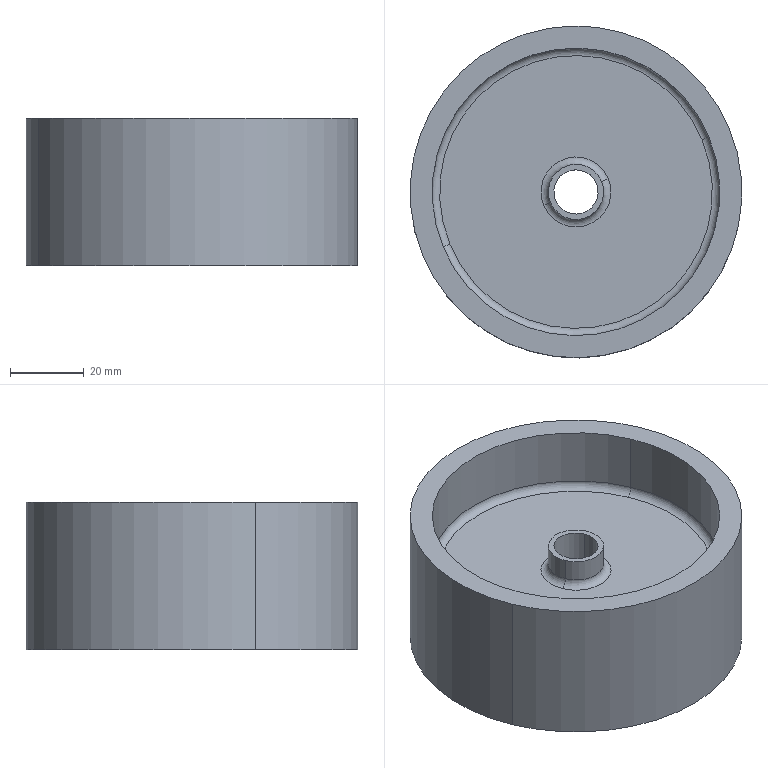Component | SolidWorks | SpringCover-2 | 1 solid | 38 faces | box 90 x 90 x 40 mm | volume 80853 mm3 | cylinder 18 | torus 12 | plane 8 | commonest cylinder face diameters 78 x4 82 x2 15 x2 86 x2 18 x2 24 x2 12 x2 90 x2
build123d program:
from build123d import *

# Parameters (mm, degrees)
SKETCH1_2_R         = 45
SKETCH1_2_R_2       = 39
BOSS_EXTRUDE1_DEPTH = 20
SKETCH2_R           = 40
SKETCH2_R_2         = 6
BOSS_EXTRUDE2_DEPTH = 2
SKETCH3_R           = 12
SKETCH3_R_2         = 9
BOSS_EXTRUDE3_DEPTH = 16
BOSS_EXTRUDE4_START = 8
SKETCH5_R           = 7.5
SKETCH5_R_2         = 6
BOSS_EXTRUDE4_DEPTH = 8
FILLET1_R           = 2
CUT_EXTRUDE1_START  = -6
SKETCH1_R           = 43
SKETCH1_R_2         = 41
CUT_EXTRUDE1_DEPTH  = 6


with BuildPart() as part:
    # Sketch1_2 → Boss-Extrude1 (new, symmetric)
    with BuildSketch(Plane.XY):
        Circle(SKETCH1_2_R)
        Circle(SKETCH1_2_R_2, mode=Mode.SUBTRACT)
    extrude(amount=BOSS_EXTRUDE1_DEPTH, both=True)

    # Sketch2 → Boss-Extrude2 (add, symmetric)
    with BuildSketch(Plane.XY):
        Circle(SKETCH2_R)
        Circle(SKETCH2_R_2, mode=Mode.SUBTRACT)
    extrude(amount=BOSS_EXTRUDE2_DEPTH, both=True)

    # Sketch3 → Boss-Extrude3 (add)
    with BuildSketch(Plane.XY.offset(2)):
        Circle(SKETCH3_R)
        Circle(SKETCH3_R_2, mode=Mode.SUBTRACT)
    extrude(amount=BOSS_EXTRUDE3_DEPTH)

    # Sketch4 → Cut-Revolve1 (revolve, cut)
    with BuildSketch(Plane(origin=(0, 0, 0), x_dir=(1, 0, 0), z_dir=(0, 1, 0))):
        Polygon((-43, -16), (-33.035, -16), (-33.287, -20), (-43, -20), align=None)
    revolve(axis=Axis((0, 0, -26.979), (0, 0, 1)), mode=Mode.SUBTRACT)

    # Sketch5 → Boss-Extrude4 (add)
    with BuildSketch(Plane(origin=(0, 0, -2), x_dir=(-1, 0, 0), z_dir=(0, 0, -1)).offset(BOSS_EXTRUDE4_START)):
        with Locations(Location((0, 0, 0), (0, 0, 180))):
            Circle(SKETCH5_R)
        Circle(SKETCH5_R_2, mode=Mode.SUBTRACT)
    extrude(amount=-BOSS_EXTRUDE4_DEPTH)

    # Fillet1
    fillet1_edges = [part.edges().sort_by_distance(p)[0] for p in [
        (-39, 0, 2),
        (-39, 0, -2),
        (-9, 0, 2),
        (-12, 0, 2),
        (-39, 0, 16),
        (-7.5, 0, -2),
    ]]
    fillet(fillet1_edges, radius=FILLET1_R)

    # Sketch1 → Cut-Extrude1 (cut)
    with BuildSketch(Plane.XY.offset(20).offset(CUT_EXTRUDE1_START)):
        with Locations(Location((0, 0, 0), (0, 0, 180))):
            Circle(SKETCH1_R)
        Circle(SKETCH1_R_2, mode=Mode.SUBTRACT)
    extrude(amount=CUT_EXTRUDE1_DEPTH, mode=Mode.SUBTRACT)


solid = part.part

# Placed as in the assembly
solid = solid.moved(Location((-15.928, -1.7, 188), (180, 0, 0)))
STEP:
#1=COLOUR_RGB('',0.7922,0.8196,0.9333);
#2=FILL_AREA_STYLE_COLOUR('',#1);
#3=FILL_AREA_STYLE('',(#2));
#4=SURFACE_STYLE_FILL_AREA(#3);
#5=SURFACE_SIDE_STYLE('',(#4));
#6=SURFACE_STYLE_USAGE(.BOTH.,#5);
#7=PRESENTATION_STYLE_ASSIGNMENT((#6));
#8=CARTESIAN_POINT('',(0.864,0.5514,6.85));
#9=VERTEX_POINT('',#8);
#10=CARTESIAN_POINT('',(-2.118,-0.6852,6.85));
#11=VERTEX_POINT('',#10);
#12=CARTESIAN_POINT('',(-0.6271,-0.06694,6.85));
#13=DIRECTION('',(0.,0.,-1.));
#14=DIRECTION('',(0.9237,0.383,0.));
#15=AXIS2_PLACEMENT_3D('',#12,#13,#14);
#16=CIRCLE('',#15,1.614);
#17=EDGE_CURVE('',#9,#11,#16,.T.);
#18=ORIENTED_EDGE('',*,*,#17,.T.);
#19=CARTESIAN_POINT('',(-2.118,-0.6852,6.772));
#20=VERTEX_POINT('',#19);
#21=CARTESIAN_POINT('',(-2.118,-0.6852,6.85));
#22=DIRECTION('',(0.,0.,-1.));
#23=VECTOR('',#22,39.37);
#24=LINE('',#21,#23);
#25=EDGE_CURVE('',#11,#20,#24,.T.);
#26=ORIENTED_EDGE('',*,*,#25,.T.);
#27=CARTESIAN_POINT('',(0.864,0.5514,6.772));
#28=VERTEX_POINT('',#27);
#29=CARTESIAN_POINT('',(-0.6271,-0.06694,6.772));
#30=DIRECTION('',(0.,0.,-1.));
#31=DIRECTION('',(-0.9237,-0.383,0.));
#32=AXIS2_PLACEMENT_3D('',#29,#30,#31);
#33=CIRCLE('',#32,1.614);
#34=EDGE_CURVE('',#28,#20,#33,.T.);
#35=ORIENTED_EDGE('',*,*,#34,.F.);
#36=CARTESIAN_POINT('',(0.864,0.5514,6.85));
#37=DIRECTION('',(0.,0.,-1.));
#38=VECTOR('',#37,39.37);
#39=LINE('',#36,#38);
#40=EDGE_CURVE('',#9,#28,#39,.T.);
#41=ORIENTED_EDGE('',*,*,#40,.F.);
#42=EDGE_LOOP('',(#18,#26,#35,#41));
#43=FACE_OUTER_BOUND('',#42,.T.);
#44=CARTESIAN_POINT('',(-0.6271,-0.06694,6.85));
#45=DIRECTION('',(0.,0.,-1.));
#46=DIRECTION('',(0.9237,0.383,0.));
#47=AXIS2_PLACEMENT_3D('',#44,#45,#46);
#48=CYLINDRICAL_SURFACE('',#47,1.614);
#49=ADVANCED_FACE('',(#43),#48,.T.);
#50=CARTESIAN_POINT('',(-1.973,-0.6249,7.323));
#51=VERTEX_POINT('',#50);
#52=CARTESIAN_POINT('',(0.7185,0.491,7.323));
#53=VERTEX_POINT('',#52);
#54=CARTESIAN_POINT('',(-0.6271,-0.06694,7.323));
#55=DIRECTION('',(0.,0.,-1.));
#56=DIRECTION('',(0.9237,0.383,0.));
#57=AXIS2_PLACEMENT_3D('',#54,#55,#56);
#58=CIRCLE('',#57,1.457);
#59=EDGE_CURVE('',#51,#53,#58,.T.);
#60=ORIENTED_EDGE('',*,*,#59,.F.);
#61=CARTESIAN_POINT('',(-2.045,-0.6551,7.244));
#62=VERTEX_POINT('',#61);
#63=CARTESIAN_POINT('',(-1.973,-0.6249,7.244));
#64=DIRECTION('',(0.383,-0.9237,0.));
#65=DIRECTION('',(0.9237,0.383,0.));
#66=AXIS2_PLACEMENT_3D('',#63,#64,#65);
#67=CIRCLE('',#66,0.07874);
#68=EDGE_CURVE('',#51,#62,#67,.T.);
#69=ORIENTED_EDGE('',*,*,#68,.T.);
#70=CARTESIAN_POINT('',(0.7912,0.5212,7.244));
#71=VERTEX_POINT('',#70);
#72=CARTESIAN_POINT('',(-0.6271,-0.06694,7.244));
#73=DIRECTION('',(0.,0.,1.));
#74=DIRECTION('',(0.9237,0.383,0.));
#75=AXIS2_PLACEMENT_3D('',#72,#73,#74);
#76=CIRCLE('',#75,1.535);
#77=EDGE_CURVE('',#71,#62,#76,.T.);
#78=ORIENTED_EDGE('',*,*,#77,.F.);
#79=CARTESIAN_POINT('',(0.7185,0.491,7.244));
#80=DIRECTION('',(-0.383,0.9237,0.));
#81=DIRECTION('',(-0.9237,-0.383,0.));
#82=AXIS2_PLACEMENT_3D('',#79,#80,#81);
#83=CIRCLE('',#82,0.07874);
#84=EDGE_CURVE('',#53,#71,#83,.T.);
#85=ORIENTED_EDGE('',*,*,#84,.F.);
#86=EDGE_LOOP('',(#60,#69,#78,#85));
#87=FACE_OUTER_BOUND('',#86,.T.);
#88=CARTESIAN_POINT('',(-0.6271,-0.06694,7.244));
#89=DIRECTION('',(0.,0.,-1.));
#90=DIRECTION('',(0.9237,0.383,0.));
#91=AXIS2_PLACEMENT_3D('',#88,#89,#90);
#92=TOROIDAL_SURFACE('',#91,1.457,0.07874);
#93=ADVANCED_FACE('',(#87),#92,.F.);
#94=CARTESIAN_POINT('',(0.7912,0.5212,6.85));
#95=VERTEX_POINT('',#94);
#96=CARTESIAN_POINT('',(-2.045,-0.6551,6.85));
#97=VERTEX_POINT('',#96);
#98=CARTESIAN_POINT('',(-0.6271,-0.06694,6.85));
#99=DIRECTION('',(0.,0.,-1.));
#100=DIRECTION('',(-0.9237,-0.383,0.));
#101=AXIS2_PLACEMENT_3D('',#98,#99,#100);
#102=CIRCLE('',#101,1.535);
#103=EDGE_CURVE('',#95,#97,#102,.T.);
#104=ORIENTED_EDGE('',*,*,#103,.F.);
#105=CARTESIAN_POINT('',(0.864,0.5514,6.85));
#106=DIRECTION('',(0.383,-0.9237,0.));
#107=DIRECTION('',(0.9237,0.383,0.));
#108=AXIS2_PLACEMENT_3D('',#105,#106,#107);
#109=CIRCLE('',#108,0.07874);
#110=EDGE_CURVE('',#95,#28,#109,.T.);
#111=ORIENTED_EDGE('',*,*,#110,.T.);
#112=ORIENTED_EDGE('',*,*,#34,.T.);
#113=CARTESIAN_POINT('',(-2.118,-0.6852,6.85));
#114=DIRECTION('',(-0.383,0.9237,0.));
#115=DIRECTION('',(-0.9237,-0.383,0.));
#116=AXIS2_PLACEMENT_3D('',#113,#114,#115);
#117=CIRCLE('',#116,0.07874);
#118=EDGE_CURVE('',#97,#20,#117,.T.);
#119=ORIENTED_EDGE('',*,*,#118,.F.);
#120=EDGE_LOOP('',(#104,#111,#112,#119));
#121=FACE_OUTER_BOUND('',#120,.T.);
#122=CARTESIAN_POINT('',(-0.6271,-0.06694,6.85));
#123=DIRECTION('',(0.,0.,1.));
#124=DIRECTION('',(-0.9237,-0.383,0.));
#125=AXIS2_PLACEMENT_3D('',#122,#123,#124);
#126=TOROIDAL_SURFACE('',#125,1.614,0.07874);
#127=ADVANCED_FACE('',(#121),#126,.T.);
#128=CARTESIAN_POINT('',(-0.8817,-0.1725,7.323));
#129=VERTEX_POINT('',#128);
#130=CARTESIAN_POINT('',(-0.3725,0.03863,7.323));
#131=VERTEX_POINT('',#130);
#132=CARTESIAN_POINT('',(-0.6271,-0.06694,7.323));
#133=DIRECTION('',(0.,0.,-1.));
#134=DIRECTION('',(0.9237,0.383,0.));
#135=AXIS2_PLACEMENT_3D('',#132,#133,#134);
#136=CIRCLE('',#135,0.2756);
#137=EDGE_CURVE('',#129,#131,#136,.T.);
#138=ORIENTED_EDGE('',*,*,#137,.F.);
#139=CARTESIAN_POINT('',(-0.9544,-0.2027,7.244));
#140=VERTEX_POINT('',#139);
#141=CARTESIAN_POINT('',(-0.8817,-0.1725,7.244));
#142=DIRECTION('',(0.383,-0.9237,0.));
#143=DIRECTION('',(0.9237,0.383,0.));
#144=AXIS2_PLACEMENT_3D('',#141,#142,#143);
#145=CIRCLE('',#144,0.07874);
#146=EDGE_CURVE('',#129,#140,#145,.T.);
#147=ORIENTED_EDGE('',*,*,#146,.T.);
#148=CARTESIAN_POINT('',(-0.2998,0.06879,7.244));
#149=VERTEX_POINT('',#148);
#150=CARTESIAN_POINT('',(-0.6271,-0.06694,7.244));
#151=DIRECTION('',(0.,0.,1.));
#152=DIRECTION('',(0.9237,0.383,0.));
#153=AXIS2_PLACEMENT_3D('',#150,#151,#152);
#154=CIRCLE('',#153,0.3543);
#155=EDGE_CURVE('',#149,#140,#154,.T.);
#156=ORIENTED_EDGE('',*,*,#155,.F.);
#157=CARTESIAN_POINT('',(-0.3725,0.03863,7.244));
#158=DIRECTION('',(-0.383,0.9237,0.));
#159=DIRECTION('',(-0.9237,-0.383,0.));
#160=AXIS2_PLACEMENT_3D('',#157,#158,#159);
#161=CIRCLE('',#160,0.07874);
#162=EDGE_CURVE('',#131,#149,#161,.T.);
#163=ORIENTED_EDGE('',*,*,#162,.F.);
#164=EDGE_LOOP('',(#138,#147,#156,#163));
#165=FACE_OUTER_BOUND('',#164,.T.);
#166=CARTESIAN_POINT('',(-0.6271,-0.06694,7.244));
#167=DIRECTION('',(0.,0.,-1.));
#168=DIRECTION('',(0.9237,0.383,0.));
#169=AXIS2_PLACEMENT_3D('',#166,#167,#168);
#170=TOROIDAL_SURFACE('',#169,0.2756,0.07874);
#171=ADVANCED_FACE('',(#165),#170,.F.);
#172=CARTESIAN_POINT('',(-1.063,-0.2479,7.244));
#173=VERTEX_POINT('',#172);
#174=CARTESIAN_POINT('',(-0.1907,0.114,7.244));
#175=VERTEX_POINT('',#174);
#176=CARTESIAN_POINT('',(-0.6271,-0.06694,7.244));
#177=DIRECTION('',(0.,0.,-1.));
#178=DIRECTION('',(0.9237,0.383,0.));
#179=AXIS2_PLACEMENT_3D('',#176,#177,#178);
#180=CIRCLE('',#179,0.4724);
#181=EDGE_CURVE('',#173,#175,#180,.T.);
#182=ORIENTED_EDGE('',*,*,#181,.F.);
#183=CARTESIAN_POINT('',(-1.136,-0.2781,7.323));
#184=VERTEX_POINT('',#183);
#185=CARTESIAN_POINT('',(-1.136,-0.2781,7.244));
#186=DIRECTION('',(0.383,-0.9237,0.));
#187=DIRECTION('',(0.9237,0.383,0.));
#188=AXIS2_PLACEMENT_3D('',#185,#186,#187);
#189=CIRCLE('',#188,0.07874);
#190=EDGE_CURVE('',#173,#184,#189,.T.);
#191=ORIENTED_EDGE('',*,*,#190,.T.);
#192=CARTESIAN_POINT('',(-0.1179,0.1442,7.323));
#193=VERTEX_POINT('',#192);
#194=CARTESIAN_POINT('',(-0.6271,-0.06694,7.323));
#195=DIRECTION('',(0.,0.,1.));
#196=DIRECTION('',(0.9237,0.383,0.));
#197=AXIS2_PLACEMENT_3D('',#194,#195,#196);
#198=CIRCLE('',#197,0.5512);
#199=EDGE_CURVE('',#193,#184,#198,.T.);
#200=ORIENTED_EDGE('',*,*,#199,.F.);
#201=CARTESIAN_POINT('',(-0.1179,0.1442,7.244));
#202=DIRECTION('',(-0.383,0.9237,0.));
#203=DIRECTION('',(-0.9237,-0.383,0.));
#204=AXIS2_PLACEMENT_3D('',#201,#202,#203);
#205=CIRCLE('',#204,0.07874);
#206=EDGE_CURVE('',#175,#193,#205,.T.);
#207=ORIENTED_EDGE('',*,*,#206,.F.);
#208=EDGE_LOOP('',(#182,#191,#200,#207));
#209=FACE_OUTER_BOUND('',#208,.T.);
#210=CARTESIAN_POINT('',(-0.6271,-0.06694,7.244));
#211=DIRECTION('',(0.,0.,-1.));
#212=DIRECTION('',(0.9237,0.383,0.));
#213=AXIS2_PLACEMENT_3D('',#210,#211,#212);
#214=TOROIDAL_SURFACE('',#213,0.5512,0.07874);
#215=ADVANCED_FACE('',(#209),#214,.F.);
#216=CARTESIAN_POINT('',(-2.045,-0.6551,7.559));
#217=VERTEX_POINT('',#216);
#218=CARTESIAN_POINT('',(0.7912,0.5212,7.559));
#219=VERTEX_POINT('',#218);
#220=CARTESIAN_POINT('',(-0.6271,-0.06694,7.559));
#221=DIRECTION('',(0.,0.,-1.));
#222=DIRECTION('',(0.9237,0.383,0.));
#223=AXIS2_PLACEMENT_3D('',#220,#221,#222);
#224=CIRCLE('',#223,1.535);
#225=EDGE_CURVE('',#217,#219,#224,.T.);
#226=ORIENTED_EDGE('',*,*,#225,.F.);
#227=CARTESIAN_POINT('',(-1.973,-0.6249,7.48));
#228=VERTEX_POINT('',#227);
#229=CARTESIAN_POINT('',(-1.973,-0.6249,7.559));
#230=DIRECTION('',(0.383,-0.9237,0.));
#231=DIRECTION('',(0.9237,0.383,0.));
#232=AXIS2_PLACEMENT_3D('',#229,#230,#231);
#233=CIRCLE('',#232,0.07874);
#234=EDGE_CURVE('',#217,#228,#233,.T.);
#235=ORIENTED_EDGE('',*,*,#234,.T.);
#236=CARTESIAN_POINT('',(0.7185,0.491,7.48));
#237=VERTEX_POINT('',#236);
#238=CARTESIAN_POINT('',(-0.6271,-0.06694,7.48));
#239=DIRECTION('',(0.,0.,1.));
#240=DIRECTION('',(0.9237,0.383,0.));
#241=AXIS2_PLACEMENT_3D('',#238,#239,#240);
#242=CIRCLE('',#241,1.457);
#243=EDGE_CURVE('',#237,#228,#242,.T.);
#244=ORIENTED_EDGE('',*,*,#243,.F.);
#245=CARTESIAN_POINT('',(0.7185,0.491,7.559));
#246=DIRECTION('',(-0.383,0.9237,0.));
#247=DIRECTION('',(-0.9237,-0.383,0.));
#248=AXIS2_PLACEMENT_3D('',#245,#246,#247);
#249=CIRCLE('',#248,0.07874);
#250=EDGE_CURVE('',#219,#237,#249,.T.);
#251=ORIENTED_EDGE('',*,*,#250,.F.);
#252=EDGE_LOOP('',(#226,#235,#244,#251));
#253=FACE_OUTER_BOUND('',#252,.T.);
#254=CARTESIAN_POINT('',(-0.6271,-0.06694,7.559));
#255=DIRECTION('',(0.,0.,-1.));
#256=DIRECTION('',(0.9237,0.383,0.));
#257=AXIS2_PLACEMENT_3D('',#254,#255,#256);
#258=TOROIDAL_SURFACE('',#257,1.457,0.07874);
#259=ADVANCED_FACE('',(#253),#258,.F.);
#260=CARTESIAN_POINT('',(-0.9726,-0.2102,7.48));
#261=VERTEX_POINT('',#260);
#262=CARTESIAN_POINT('',(-0.2816,0.07633,7.48));
#263=VERTEX_POINT('',#262);
#264=CARTESIAN_POINT('',(-0.6271,-0.06694,7.48));
#265=DIRECTION('',(0.,0.,-1.));
#266=DIRECTION('',(0.9237,0.383,0.));
#267=AXIS2_PLACEMENT_3D('',#264,#265,#266);
#268=CIRCLE('',#267,0.374);
#269=EDGE_CURVE('',#261,#263,#268,.T.);
#270=ORIENTED_EDGE('',*,*,#269,.F.);
#271=CARTESIAN_POINT('',(-0.8998,-0.18,7.559));
#272=VERTEX_POINT('',#271);
#273=CARTESIAN_POINT('',(-0.9726,-0.2102,7.559));
#274=DIRECTION('',(0.383,-0.9237,0.));
#275=DIRECTION('',(0.9237,0.383,0.));
#276=AXIS2_PLACEMENT_3D('',#273,#274,#275);
#277=CIRCLE('',#276,0.07874);
#278=EDGE_CURVE('',#261,#272,#277,.T.);
#279=ORIENTED_EDGE('',*,*,#278,.T.);
#280=CARTESIAN_POINT('',(-0.3543,0.04617,7.559));
#281=VERTEX_POINT('',#280);
#282=CARTESIAN_POINT('',(-0.6271,-0.06694,7.559));
#283=DIRECTION('',(0.,0.,1.));
#284=DIRECTION('',(0.9237,0.383,0.));
#285=AXIS2_PLACEMENT_3D('',#282,#283,#284);
#286=CIRCLE('',#285,0.2953);
#287=EDGE_CURVE('',#281,#272,#286,.T.);
#288=ORIENTED_EDGE('',*,*,#287,.F.);
#289=CARTESIAN_POINT('',(-0.2816,0.07633,7.559));
#290=DIRECTION('',(-0.383,0.9237,0.));
#291=DIRECTION('',(-0.9237,-0.383,0.));
#292=AXIS2_PLACEMENT_3D('',#289,#290,#291);
#293=CIRCLE('',#292,0.07874);
#294=EDGE_CURVE('',#263,#281,#293,.T.);
#295=ORIENTED_EDGE('',*,*,#294,.F.);
#296=EDGE_LOOP('',(#270,#279,#288,#295));
#297=FACE_OUTER_BOUND('',#296,.T.);
#298=CARTESIAN_POINT('',(-0.6271,-0.06694,7.559));
#299=DIRECTION('',(0.,0.,-1.));
#300=DIRECTION('',(0.9237,0.383,0.));
#301=AXIS2_PLACEMENT_3D('',#298,#299,#300);
#302=TOROIDAL_SURFACE('',#301,0.374,0.07874);
#303=ADVANCED_FACE('',(#297),#302,.F.);
#304=CARTESIAN_POINT('',(-0.8998,-0.18,7.795));
#305=VERTEX_POINT('',#304);
#306=CARTESIAN_POINT('',(-0.3543,0.04617,7.795));
#307=VERTEX_POINT('',#306);
#308=CARTESIAN_POINT('',(-0.6271,-0.06694,7.795));
#309=DIRECTION('',(0.,0.,1.));
#310=DIRECTION('',(-0.9237,-0.383,0.));
#311=AXIS2_PLACEMENT_3D('',#308,#309,#310);
#312=CIRCLE('',#311,0.2953);
#313=EDGE_CURVE('',#305,#307,#312,.T.);
#314=ORIENTED_EDGE('',*,*,#313,.F.);
#315=CARTESIAN_POINT('',(-0.8998,-0.18,7.795));
#316=DIRECTION('',(0.,0.,-1.));
#317=VECTOR('',#316,39.37);
#318=LINE('',#315,#317);
#319=EDGE_CURVE('',#305,#272,#318,.T.);
#320=ORIENTED_EDGE('',*,*,#319,.T.);
#321=CARTESIAN_POINT('',(-0.6271,-0.06694,7.559));
#322=DIRECTION('',(0.,0.,1.));
#323=DIRECTION('',(0.9237,0.383,0.));
#324=AXIS2_PLACEMENT_3D('',#321,#322,#323);
#325=CIRCLE('',#324,0.2953);
#326=EDGE_CURVE('',#272,#281,#325,.T.);
#327=ORIENTED_EDGE('',*,*,#326,.T.);
#328=CARTESIAN_POINT('',(-0.3543,0.04617,7.795));
#329=DIRECTION('',(0.,0.,-1.));
#330=VECTOR('',#329,39.37);
#331=LINE('',#328,#330);
#332=EDGE_CURVE('',#307,#281,#331,.T.);
#333=ORIENTED_EDGE('',*,*,#332,.F.);
#334=EDGE_LOOP('',(#314,#320,#327,#333));
#335=FACE_OUTER_BOUND('',#334,.T.);
#336=CARTESIAN_POINT('',(-0.6271,-0.06694,7.795));
#337=DIRECTION('',(0.,0.,-1.));
#338=DIRECTION('',(0.9237,0.383,0.));
#339=AXIS2_PLACEMENT_3D('',#336,#337,#338);
#340=CYLINDRICAL_SURFACE('',#339,0.2953);
#341=ADVANCED_FACE('',(#335),#340,.T.);
#342=CARTESIAN_POINT('',(0.9367,0.5815,6.614));
#343=VERTEX_POINT('',#342);
#344=CARTESIAN_POINT('',(-2.191,-0.7154,6.614));
#345=VERTEX_POINT('',#344);
#346=CARTESIAN_POINT('',(-0.6271,-0.06694,6.614));
#347=DIRECTION('',(0.,0.,1.));
#348=DIRECTION('',(-0.9237,-0.383,0.));
#349=AXIS2_PLACEMENT_3D('',#346,#347,#348);
#350=CIRCLE('',#349,1.693);
#351=EDGE_CURVE('',#343,#345,#350,.T.);
#352=ORIENTED_EDGE('',*,*,#351,.F.);
#353=CARTESIAN_POINT('',(0.9367,0.5815,6.85));
#354=VERTEX_POINT('',#353);
#355=CARTESIAN_POINT('',(0.9367,0.5815,8.464));
#356=DIRECTION('',(0.,0.,1.));
#357=VECTOR('',#356,39.37);
#358=LINE('',#355,#357);
#359=EDGE_CURVE('',#343,#354,#358,.T.);
#360=ORIENTED_EDGE('',*,*,#359,.T.);
#361=CARTESIAN_POINT('',(-2.191,-0.7154,6.85));
#362=VERTEX_POINT('',#361);
#363=CARTESIAN_POINT('',(-0.6271,-0.06694,6.85));
#364=DIRECTION('',(0.,0.,-1.));
#365=DIRECTION('',(0.9237,0.383,0.));
#366=AXIS2_PLACEMENT_3D('',#363,#364,#365);
#367=CIRCLE('',#366,1.693);
#368=EDGE_CURVE('',#362,#354,#367,.T.);
#369=ORIENTED_EDGE('',*,*,#368,.F.);
#370=CARTESIAN_POINT('',(-2.191,-0.7154,8.464));
#371=DIRECTION('',(0.,0.,1.));
#372=VECTOR('',#371,39.37);
#373=LINE('',#370,#372);
#374=EDGE_CURVE('',#345,#362,#373,.T.);
#375=ORIENTED_EDGE('',*,*,#374,.F.);
#376=EDGE_LOOP('',(#352,#360,#369,#375));
#377=FACE_OUTER_BOUND('',#376,.T.);
#378=CARTESIAN_POINT('',(-0.6271,-0.06694,8.464));
#379=DIRECTION('',(0.,0.,1.));
#380=DIRECTION('',(-0.9237,-0.383,0.));
#381=AXIS2_PLACEMENT_3D('',#378,#379,#380);
#382=CYLINDRICAL_SURFACE('',#381,1.693);
#383=ADVANCED_FACE('',(#377),#382,.F.);
#384=CARTESIAN_POINT('',(-0.9544,-0.2027,6.693));
#385=VERTEX_POINT('',#384);
#386=CARTESIAN_POINT('',(-0.2998,0.06879,6.693));
#387=VERTEX_POINT('',#386);
#388=CARTESIAN_POINT('',(-0.6271,-0.06694,6.693));
#389=DIRECTION('',(0.,0.,-1.));
#390=DIRECTION('',(0.9237,0.383,0.));
#391=AXIS2_PLACEMENT_3D('',#388,#389,#390);
#392=CIRCLE('',#391,0.3543);
#393=EDGE_CURVE('',#385,#387,#392,.T.);
#394=ORIENTED_EDGE('',*,*,#393,.T.);
#395=CARTESIAN_POINT('',(-0.2998,0.06879,6.693));
#396=DIRECTION('',(0.,0.,1.));
#397=VECTOR('',#396,39.37);
#398=LINE('',#395,#397);
#399=EDGE_CURVE('',#387,#149,#398,.T.);
#400=ORIENTED_EDGE('',*,*,#399,.T.);
#401=ORIENTED_EDGE('',*,*,#155,.T.);
#402=CARTESIAN_POINT('',(-0.9544,-0.2027,6.693));
#403=DIRECTION('',(0.,0.,1.));
#404=VECTOR('',#403,39.37);
#405=LINE('',#402,#404);
#406=EDGE_CURVE('',#385,#140,#405,.T.);
#407=ORIENTED_EDGE('',*,*,#406,.F.);
#408=EDGE_LOOP('',(#394,#400,#401,#407));
#409=FACE_OUTER_BOUND('',#408,.T.);
#410=CARTESIAN_POINT('',(-0.6271,-0.06694,6.693));
#411=DIRECTION('',(0.,0.,1.));
#412=DIRECTION('',(-0.9237,-0.383,0.));
#413=AXIS2_PLACEMENT_3D('',#410,#411,#412);
#414=CYLINDRICAL_SURFACE('',#413,0.3543);
#415=ADVANCED_FACE('',(#409),#414,.F.);
#416=CARTESIAN_POINT('',(-0.1907,0.114,6.693));
#417=VERTEX_POINT('',#416);
#418=CARTESIAN_POINT('',(-1.063,-0.2479,6.693));
#419=VERTEX_POINT('',#418);
#420=CARTESIAN_POINT('',(-0.6271,-0.06694,6.693));
#421=DIRECTION('',(0.,0.,-1.));
#422=DIRECTION('',(0.9237,0.383,0.));
#423=AXIS2_PLACEMENT_3D('',#420,#421,#422);
#424=CIRCLE('',#423,0.4724);
#425=EDGE_CURVE('',#417,#419,#424,.T.);
#426=ORIENTED_EDGE('',*,*,#425,.F.);
#427=CARTESIAN_POINT('',(-0.1907,0.114,6.693));
#428=DIRECTION('',(0.,0.,1.));
#429=VECTOR('',#428,39.37);
#430=LINE('',#427,#429);
#431=EDGE_CURVE('',#417,#175,#430,.T.);
#432=ORIENTED_EDGE('',*,*,#431,.T.);
#433=CARTESIAN_POINT('',(-0.6271,-0.06694,7.244));
#434=DIRECTION('',(0.,0.,-1.));
#435=DIRECTION('',(0.9237,0.383,0.));
#436=AXIS2_PLACEMENT_3D('',#433,#434,#435);
#437=CIRCLE('',#436,0.4724);
#438=EDGE_CURVE('',#175,#173,#437,.T.);
#439=ORIENTED_EDGE('',*,*,#438,.T.);
#440=CARTESIAN_POINT('',(-1.063,-0.2479,6.693));
#441=DIRECTION('',(0.,0.,1.));
#442=VECTOR('',#441,39.37);
#443=LINE('',#440,#442);
#444=EDGE_CURVE('',#419,#173,#443,.T.);
#445=ORIENTED_EDGE('',*,*,#444,.F.);
#446=EDGE_LOOP('',(#426,#432,#439,#445));
#447=FACE_OUTER_BOUND('',#446,.T.);
#448=CARTESIAN_POINT('',(-0.6271,-0.06694,6.693));
#449=DIRECTION('',(0.,0.,1.));
#450=DIRECTION('',(-0.9237,-0.383,0.));
#451=AXIS2_PLACEMENT_3D('',#448,#449,#450);
#452=CYLINDRICAL_SURFACE('',#451,0.4724);
#453=ADVANCED_FACE('',(#447),#452,.T.);
#454=CARTESIAN_POINT('',(-0.8453,-0.1574,7.323));
#455=VERTEX_POINT('',#454);
#456=CARTESIAN_POINT('',(-0.4089,0.02355,7.323));
#457=VERTEX_POINT('',#456);
#458=CARTESIAN_POINT('',(-0.6271,-0.06694,7.323));
#459=DIRECTION('',(0.,0.,-1.));
#460=DIRECTION('',(0.9237,0.383,0.));
#461=AXIS2_PLACEMENT_3D('',#458,#459,#460);
#462=CIRCLE('',#461,0.2362);
#463=EDGE_CURVE('',#455,#457,#462,.T.);
#464=ORIENTED_EDGE('',*,*,#463,.T.);
#465=CARTESIAN_POINT('',(-0.4089,0.02355,7.795));
#466=VERTEX_POINT('',#465);
#467=CARTESIAN_POINT('',(-0.4089,0.02355,7.323));
#468=DIRECTION('',(0.,0.,1.));
#469=VECTOR('',#468,39.37);
#470=LINE('',#467,#469);
#471=EDGE_CURVE('',#457,#466,#470,.T.);
#472=ORIENTED_EDGE('',*,*,#471,.T.);
#473=CARTESIAN_POINT('',(-0.8453,-0.1574,7.795));
#474=VERTEX_POINT('',#473);
#475=CARTESIAN_POINT('',(-0.6271,-0.06694,7.795));
#476=DIRECTION('',(0.,0.,1.));
#477=DIRECTION('',(-0.9237,-0.383,0.));
#478=AXIS2_PLACEMENT_3D('',#475,#476,#477);
#479=CIRCLE('',#478,0.2362);
#480=EDGE_CURVE('',#466,#474,#479,.T.);
#481=ORIENTED_EDGE('',*,*,#480,.T.);
#482=CARTESIAN_POINT('',(-0.8453,-0.1574,7.323));
#483=DIRECTION('',(0.,0.,1.));
#484=VECTOR('',#483,39.37);
#485=LINE('',#482,#484);
#486=EDGE_CURVE('',#455,#474,#485,.T.);
#487=ORIENTED_EDGE('',*,*,#486,.F.);
#488=EDGE_LOOP('',(#464,#472,#481,#487));
#489=FACE_OUTER_BOUND('',#488,.T.);
#490=CARTESIAN_POINT('',(-0.6271,-0.06694,7.323));
#491=DIRECTION('',(0.,0.,1.));
#492=DIRECTION('',(-0.9237,-0.383,0.));
#493=AXIS2_PLACEMENT_3D('',#490,#491,#492);
#494=CYLINDRICAL_SURFACE('',#493,0.2362);
#495=ADVANCED_FACE('',(#489),#494,.F.);
#496=CARTESIAN_POINT('',(-0.6271,-0.06694,6.85));
#497=DIRECTION('',(0.,0.,-1.));
#498=DIRECTION('',(-0.9237,-0.383,0.));
#499=AXIS2_PLACEMENT_3D('',#496,#497,#498);
#500=CIRCLE('',#499,1.535);
#501=EDGE_CURVE('',#97,#95,#500,.T.);
#502=ORIENTED_EDGE('',*,*,#501,.T.);
#503=CARTESIAN_POINT('',(0.7912,0.5212,6.614));
#504=DIRECTION('',(0.,0.,1.));
#505=VECTOR('',#504,39.37);
#506=LINE('',#503,#505);
#507=EDGE_CURVE('',#95,#71,#506,.T.);
#508=ORIENTED_EDGE('',*,*,#507,.T.);
#509=ORIENTED_EDGE('',*,*,#77,.T.);
#510=CARTESIAN_POINT('',(-2.045,-0.6551,6.614));
#511=DIRECTION('',(0.,0.,1.));
#512=VECTOR('',#511,39.37);
#513=LINE('',#510,#512);
#514=EDGE_CURVE('',#97,#62,#513,.T.);
#515=ORIENTED_EDGE('',*,*,#514,.F.);
#516=EDGE_LOOP('',(#502,#508,#509,#515));
#517=FACE_OUTER_BOUND('',#516,.T.);
#518=CARTESIAN_POINT('',(-0.6271,-0.06694,6.614));
#519=DIRECTION('',(0.,0.,1.));
#520=DIRECTION('',(-0.9237,-0.383,0.));
#521=AXIS2_PLACEMENT_3D('',#518,#519,#520);
#522=CYLINDRICAL_SURFACE('',#521,1.535);
#523=ADVANCED_FACE('',(#517),#522,.F.);
#524=CARTESIAN_POINT('',(1.009,0.6117,6.614));
#525=VERTEX_POINT('',#524);
#526=CARTESIAN_POINT('',(-2.264,-0.7456,6.614));
#527=VERTEX_POINT('',#526);
#528=CARTESIAN_POINT('',(-0.6271,-0.06694,6.614));
#529=DIRECTION('',(0.,0.,-1.));
#530=DIRECTION('',(0.9237,0.383,0.));
#531=AXIS2_PLACEMENT_3D('',#528,#529,#530);
#532=CIRCLE('',#531,1.772);
#533=EDGE_CURVE('',#525,#527,#532,.T.);
#534=ORIENTED_EDGE('',*,*,#533,.F.);
#535=CARTESIAN_POINT('',(1.009,0.6117,8.189));
#536=VERTEX_POINT('',#535);
#537=CARTESIAN_POINT('',(1.009,0.6117,6.614));
#538=DIRECTION('',(0.,0.,1.));
#539=VECTOR('',#538,39.37);
#540=LINE('',#537,#539);
#541=EDGE_CURVE('',#525,#536,#540,.T.);
#542=ORIENTED_EDGE('',*,*,#541,.T.);
#543=CARTESIAN_POINT('',(-2.264,-0.7456,8.189));
#544=VERTEX_POINT('',#543);
#545=CARTESIAN_POINT('',(-0.6271,-0.06694,8.189));
#546=DIRECTION('',(0.,0.,-1.));
#547=DIRECTION('',(0.9237,0.383,0.));
#548=AXIS2_PLACEMENT_3D('',#545,#546,#547);
#549=CIRCLE('',#548,1.772);
#550=EDGE_CURVE('',#536,#544,#549,.T.);
#551=ORIENTED_EDGE('',*,*,#550,.T.);
#552=CARTESIAN_POINT('',(-2.264,-0.7456,6.614));
#553=DIRECTION('',(0.,0.,1.));
#554=VECTOR('',#553,39.37);
#555=LINE('',#552,#554);
#556=EDGE_CURVE('',#527,#544,#555,.T.);
#557=ORIENTED_EDGE('',*,*,#556,.F.);
#558=EDGE_LOOP('',(#534,#542,#551,#557));
#559=FACE_OUTER_BOUND('',#558,.T.);
#560=CARTESIAN_POINT('',(-0.6271,-0.06694,6.614));
#561=DIRECTION('',(0.,0.,1.));
#562=DIRECTION('',(-0.9237,-0.383,0.));
#563=AXIS2_PLACEMENT_3D('',#560,#561,#562);
#564=CYLINDRICAL_SURFACE('',#563,1.772);
#565=ADVANCED_FACE('',(#559),#564,.T.);
#566=ORIENTED_EDGE('',*,*,#225,.T.);
#567=CARTESIAN_POINT('',(0.7912,0.5212,8.189));
#568=VERTEX_POINT('',#567);
#569=CARTESIAN_POINT('',(0.7912,0.5212,6.614));
#570=DIRECTION('',(0.,0.,1.));
#571=VECTOR('',#570,39.37);
#572=LINE('',#569,#571);
#573=EDGE_CURVE('',#219,#568,#572,.T.);
#574=ORIENTED_EDGE('',*,*,#573,.T.);
#575=CARTESIAN_POINT('',(-2.045,-0.6551,8.189));
#576=VERTEX_POINT('',#575);
#577=CARTESIAN_POINT('',(-0.6271,-0.06694,8.189));
#578=DIRECTION('',(0.,0.,-1.));
#579=DIRECTION('',(0.9237,0.383,0.));
#580=AXIS2_PLACEMENT_3D('',#577,#578,#579);
#581=CIRCLE('',#580,1.535);
#582=EDGE_CURVE('',#576,#568,#581,.T.);
#583=ORIENTED_EDGE('',*,*,#582,.F.);
#584=CARTESIAN_POINT('',(-2.045,-0.6551,6.614));
#585=DIRECTION('',(0.,0.,1.));
#586=VECTOR('',#585,39.37);
#587=LINE('',#584,#586);
#588=EDGE_CURVE('',#217,#576,#587,.T.);
#589=ORIENTED_EDGE('',*,*,#588,.F.);
#590=EDGE_LOOP('',(#566,#574,#583,#589));
#591=FACE_OUTER_BOUND('',#590,.T.);
#592=CARTESIAN_POINT('',(-0.6271,-0.06694,6.614));
#593=DIRECTION('',(0.,0.,1.));
#594=DIRECTION('',(-0.9237,-0.383,0.));
#595=AXIS2_PLACEMENT_3D('',#592,#593,#594);
#596=CYLINDRICAL_SURFACE('',#595,1.535);
#597=ADVANCED_FACE('',(#591),#596,.F.);
#598=CARTESIAN_POINT('',(-0.6271,-0.06694,7.48));
#599=DIRECTION('',(0.,0.,-1.));
#600=DIRECTION('',(0.9237,0.383,0.));
#601=AXIS2_PLACEMENT_3D('',#598,#599,#600);
#602=CIRCLE('',#601,0.374);
#603=EDGE_CURVE('',#263,#261,#602,.T.);
#604=ORIENTED_EDGE('',*,*,#603,.T.);
#605=ORIENTED_EDGE('',*,*,#269,.T.);
#606=EDGE_LOOP('',(#604,#605));
#607=FACE_BOUND('',#606,.T.);
#608=ORIENTED_EDGE('',*,*,#243,.T.);
#609=CARTESIAN_POINT('',(-0.6271,-0.06694,7.48));
#610=DIRECTION('',(0.,0.,1.));
#611=DIRECTION('',(0.9237,0.383,0.));
#612=AXIS2_PLACEMENT_3D('',#609,#610,#611);
#613=CIRCLE('',#612,1.457);
#614=EDGE_CURVE('',#228,#237,#613,.T.);
#615=ORIENTED_EDGE('',*,*,#614,.T.);
#616=EDGE_LOOP('',(#608,#615));
#617=FACE_OUTER_BOUND('',#616,.T.);
#618=CARTESIAN_POINT('',(-0.6271,-0.06694,7.48));
#619=DIRECTION('',(0.,0.,-1.));
#620=DIRECTION('',(0.9237,0.383,0.));
#621=AXIS2_PLACEMENT_3D('',#618,#619,#620);
#622=PLANE('',#621);
#623=ADVANCED_FACE('',(#607,#617),#622,.F.);
#624=ORIENTED_EDGE('',*,*,#199,.T.);
#625=CARTESIAN_POINT('',(-0.6271,-0.06694,7.323));
#626=DIRECTION('',(0.,0.,1.));
#627=DIRECTION('',(0.9237,0.383,0.));
#628=AXIS2_PLACEMENT_3D('',#625,#626,#627);
#629=CIRCLE('',#628,0.5512);
#630=EDGE_CURVE('',#184,#193,#629,.T.);
#631=ORIENTED_EDGE('',*,*,#630,.T.);
#632=EDGE_LOOP('',(#624,#631));
#633=FACE_BOUND('',#632,.T.);
#634=CARTESIAN_POINT('',(-0.6271,-0.06694,7.323));
#635=DIRECTION('',(0.,0.,-1.));
#636=DIRECTION('',(0.9237,0.383,0.));
#637=AXIS2_PLACEMENT_3D('',#634,#635,#636);
#638=CIRCLE('',#637,1.457);
#639=EDGE_CURVE('',#53,#51,#638,.T.);
#640=ORIENTED_EDGE('',*,*,#639,.T.);
#641=ORIENTED_EDGE('',*,*,#59,.T.);
#642=EDGE_LOOP('',(#640,#641));
#643=FACE_OUTER_BOUND('',#642,.T.);
#644=CARTESIAN_POINT('',(-0.6271,-0.06694,7.323));
#645=DIRECTION('',(0.,0.,-1.));
#646=DIRECTION('',(0.9237,0.383,0.));
#647=AXIS2_PLACEMENT_3D('',#644,#645,#646);
#648=PLANE('',#647);
#649=ADVANCED_FACE('',(#633,#643),#648,.T.);
#650=ORIENTED_EDGE('',*,*,#573,.F.);
#651=CARTESIAN_POINT('',(-0.6271,-0.06694,7.559));
#652=DIRECTION('',(0.,0.,-1.));
#653=DIRECTION('',(0.9237,0.383,0.));
#654=AXIS2_PLACEMENT_3D('',#651,#652,#653);
#655=CIRCLE('',#654,1.535);
#656=EDGE_CURVE('',#219,#217,#655,.T.);
#657=ORIENTED_EDGE('',*,*,#656,.T.);
#658=ORIENTED_EDGE('',*,*,#588,.T.);
#659=CARTESIAN_POINT('',(-0.6271,-0.06694,8.189));
#660=DIRECTION('',(0.,0.,-1.));
#661=DIRECTION('',(0.9237,0.383,0.));
#662=AXIS2_PLACEMENT_3D('',#659,#660,#661);
#663=CIRCLE('',#662,1.535);
#664=EDGE_CURVE('',#568,#576,#663,.T.);
#665=ORIENTED_EDGE('',*,*,#664,.F.);
#666=EDGE_LOOP('',(#650,#657,#658,#665));
#667=FACE_OUTER_BOUND('',#666,.T.);
#668=CARTESIAN_POINT('',(-0.6271,-0.06694,6.614));
#669=DIRECTION('',(0.,0.,1.));
#670=DIRECTION('',(-0.9237,-0.383,0.));
#671=AXIS2_PLACEMENT_3D('',#668,#669,#670);
#672=CYLINDRICAL_SURFACE('',#671,1.535);
#673=ADVANCED_FACE('',(#667),#672,.F.);
#674=CARTESIAN_POINT('',(-0.6271,-0.06694,6.614));
#675=DIRECTION('',(0.,0.,1.));
#676=DIRECTION('',(-0.9237,-0.383,0.));
#677=AXIS2_PLACEMENT_3D('',#674,#675,#676);
#678=CIRCLE('',#677,1.693);
#679=EDGE_CURVE('',#345,#343,#678,.T.);
#680=ORIENTED_EDGE('',*,*,#679,.T.);
#681=ORIENTED_EDGE('',*,*,#351,.T.);
#682=EDGE_LOOP('',(#680,#681));
#683=FACE_BOUND('',#682,.T.);
#684=CARTESIAN_POINT('',(-0.6271,-0.06694,6.614));
#685=DIRECTION('',(0.,0.,-1.));
#686=DIRECTION('',(0.9237,0.383,0.));
#687=AXIS2_PLACEMENT_3D('',#684,#685,#686);
#688=CIRCLE('',#687,1.772);
#689=EDGE_CURVE('',#527,#525,#688,.T.);
#690=ORIENTED_EDGE('',*,*,#689,.T.);
#691=ORIENTED_EDGE('',*,*,#533,.T.);
#692=EDGE_LOOP('',(#690,#691));
#693=FACE_OUTER_BOUND('',#692,.T.);
#694=CARTESIAN_POINT('',(-0.6271,-0.06694,6.614));
#695=DIRECTION('',(0.,0.,-1.));
#696=DIRECTION('',(0.9237,0.383,0.));
#697=AXIS2_PLACEMENT_3D('',#694,#695,#696);
#698=PLANE('',#697);
#699=ADVANCED_FACE('',(#683,#693),#698,.T.);
#700=CARTESIAN_POINT('',(-0.6271,-0.06694,8.189));
#701=DIRECTION('',(0.,0.,-1.));
#702=DIRECTION('',(0.9237,0.383,0.));
#703=AXIS2_PLACEMENT_3D('',#700,#701,#702);
#704=CIRCLE('',#703,1.772);
#705=EDGE_CURVE('',#544,#536,#704,.T.);
#706=ORIENTED_EDGE('',*,*,#705,.F.);
#707=ORIENTED_EDGE('',*,*,#550,.F.);
#708=EDGE_LOOP('',(#706,#707));
#709=FACE_OUTER_BOUND('',#708,.T.);
#710=ORIENTED_EDGE('',*,*,#582,.T.);
#711=ORIENTED_EDGE('',*,*,#664,.T.);
#712=EDGE_LOOP('',(#710,#711));
#713=FACE_BOUND('',#712,.T.);
#714=CARTESIAN_POINT('',(-0.6271,-0.06694,8.189));
#715=DIRECTION('',(0.,0.,-1.));
#716=DIRECTION('',(0.9237,0.383,0.));
#717=AXIS2_PLACEMENT_3D('',#714,#715,#716);
#718=PLANE('',#717);
#719=ADVANCED_FACE('',(#709,#713),#718,.F.);
#720=ORIENTED_EDGE('',*,*,#541,.F.);
#721=ORIENTED_EDGE('',*,*,#689,.F.);
#722=ORIENTED_EDGE('',*,*,#556,.T.);
#723=ORIENTED_EDGE('',*,*,#705,.T.);
#724=EDGE_LOOP('',(#720,#721,#722,#723));
#725=FACE_OUTER_BOUND('',#724,.T.);
#726=CARTESIAN_POINT('',(-0.6271,-0.06694,6.614));
#727=DIRECTION('',(0.,0.,1.));
#728=DIRECTION('',(-0.9237,-0.383,0.));
#729=AXIS2_PLACEMENT_3D('',#726,#727,#728);
#730=CYLINDRICAL_SURFACE('',#729,1.772);
#731=ADVANCED_FACE('',(#725),#730,.T.);
#732=ORIENTED_EDGE('',*,*,#507,.F.);
#733=ORIENTED_EDGE('',*,*,#103,.T.);
#734=ORIENTED_EDGE('',*,*,#514,.T.);
#735=CARTESIAN_POINT('',(-0.6271,-0.06694,7.244));
#736=DIRECTION('',(0.,0.,1.));
#737=DIRECTION('',(0.9237,0.383,0.));
#738=AXIS2_PLACEMENT_3D('',#735,#736,#737);
#739=CIRCLE('',#738,1.535);
#740=EDGE_CURVE('',#62,#71,#739,.T.);
#741=ORIENTED_EDGE('',*,*,#740,.T.);
#742=EDGE_LOOP('',(#732,#733,#734,#741));
#743=FACE_OUTER_BOUND('',#742,.T.);
#744=CARTESIAN_POINT('',(-0.6271,-0.06694,6.614));
#745=DIRECTION('',(0.,0.,1.));
#746=DIRECTION('',(-0.9237,-0.383,0.));
#747=AXIS2_PLACEMENT_3D('',#744,#745,#746);
#748=CYLINDRICAL_SURFACE('',#747,1.535);
#749=ADVANCED_FACE('',(#743),#748,.F.);
#750=CARTESIAN_POINT('',(-0.6271,-0.06694,7.323));
#751=DIRECTION('',(0.,0.,-1.));
#752=DIRECTION('',(0.9237,0.383,0.));
#753=AXIS2_PLACEMENT_3D('',#750,#751,#752);
#754=CIRCLE('',#753,0.2756);
#755=EDGE_CURVE('',#131,#129,#754,.T.);
#756=ORIENTED_EDGE('',*,*,#755,.T.);
#757=ORIENTED_EDGE('',*,*,#137,.T.);
#758=EDGE_LOOP('',(#756,#757));
#759=FACE_OUTER_BOUND('',#758,.T.);
#760=ORIENTED_EDGE('',*,*,#463,.F.);
#761=CARTESIAN_POINT('',(-0.6271,-0.06694,7.323));
#762=DIRECTION('',(0.,0.,-1.));
#763=DIRECTION('',(0.9237,0.383,0.));
#764=AXIS2_PLACEMENT_3D('',#761,#762,#763);
#765=CIRCLE('',#764,0.2362);
#766=EDGE_CURVE('',#457,#455,#765,.T.);
#767=ORIENTED_EDGE('',*,*,#766,.F.);
#768=EDGE_LOOP('',(#760,#767));
#769=FACE_BOUND('',#768,.T.);
#770=CARTESIAN_POINT('',(-0.6271,-0.06694,7.323));
#771=DIRECTION('',(0.,0.,-1.));
#772=DIRECTION('',(0.9237,0.383,0.));
#773=AXIS2_PLACEMENT_3D('',#770,#771,#772);
#774=PLANE('',#773);
#775=ADVANCED_FACE('',(#759,#769),#774,.T.);
#776=ORIENTED_EDGE('',*,*,#471,.F.);
#777=ORIENTED_EDGE('',*,*,#766,.T.);
#778=ORIENTED_EDGE('',*,*,#486,.T.);
#779=CARTESIAN_POINT('',(-0.6271,-0.06694,7.795));
#780=DIRECTION('',(0.,0.,1.));
#781=DIRECTION('',(-0.9237,-0.383,0.));
#782=AXIS2_PLACEMENT_3D('',#779,#780,#781);
#783=CIRCLE('',#782,0.2362);
#784=EDGE_CURVE('',#474,#466,#783,.T.);
#785=ORIENTED_EDGE('',*,*,#784,.T.);
#786=EDGE_LOOP('',(#776,#777,#778,#785));
#787=FACE_OUTER_BOUND('',#786,.T.);
#788=CARTESIAN_POINT('',(-0.6271,-0.06694,7.323));
#789=DIRECTION('',(0.,0.,1.));
#790=DIRECTION('',(-0.9237,-0.383,0.));
#791=AXIS2_PLACEMENT_3D('',#788,#789,#790);
#792=CYLINDRICAL_SURFACE('',#791,0.2362);
#793=ADVANCED_FACE('',(#787),#792,.F.);
#794=CARTESIAN_POINT('',(-0.6271,-0.06694,6.693));
#795=DIRECTION('',(0.,0.,-1.));
#796=DIRECTION('',(0.9237,0.383,0.));
#797=AXIS2_PLACEMENT_3D('',#794,#795,#796);
#798=CIRCLE('',#797,0.4724);
#799=EDGE_CURVE('',#419,#417,#798,.T.);
#800=ORIENTED_EDGE('',*,*,#799,.T.);
#801=ORIENTED_EDGE('',*,*,#425,.T.);
#802=EDGE_LOOP('',(#800,#801));
#803=FACE_OUTER_BOUND('',#802,.T.);
#804=ORIENTED_EDGE('',*,*,#393,.F.);
#805=CARTESIAN_POINT('',(-0.6271,-0.06694,6.693));
#806=DIRECTION('',(0.,0.,-1.));
#807=DIRECTION('',(0.9237,0.383,0.));
#808=AXIS2_PLACEMENT_3D('',#805,#806,#807);
#809=CIRCLE('',#808,0.3543);
#810=EDGE_CURVE('',#387,#385,#809,.T.);
#811=ORIENTED_EDGE('',*,*,#810,.F.);
#812=EDGE_LOOP('',(#804,#811));
#813=FACE_BOUND('',#812,.T.);
#814=CARTESIAN_POINT('',(-0.6271,-0.06694,6.693));
#815=DIRECTION('',(0.,0.,-1.));
#816=DIRECTION('',(0.9237,0.383,0.));
#817=AXIS2_PLACEMENT_3D('',#814,#815,#816);
#818=PLANE('',#817);
#819=ADVANCED_FACE('',(#803,#813),#818,.T.);
#820=ORIENTED_EDGE('',*,*,#431,.F.);
#821=ORIENTED_EDGE('',*,*,#799,.F.);
#822=ORIENTED_EDGE('',*,*,#444,.T.);
#823=ORIENTED_EDGE('',*,*,#181,.T.);
#824=EDGE_LOOP('',(#820,#821,#822,#823));
#825=FACE_OUTER_BOUND('',#824,.T.);
#826=CARTESIAN_POINT('',(-0.6271,-0.06694,6.693));
#827=DIRECTION('',(0.,0.,1.));
#828=DIRECTION('',(-0.9237,-0.383,0.));
#829=AXIS2_PLACEMENT_3D('',#826,#827,#828);
#830=CYLINDRICAL_SURFACE('',#829,0.4724);
#831=ADVANCED_FACE('',(#825),#830,.T.);
#832=ORIENTED_EDGE('',*,*,#399,.F.);
#833=ORIENTED_EDGE('',*,*,#810,.T.);
#834=ORIENTED_EDGE('',*,*,#406,.T.);
#835=CARTESIAN_POINT('',(-0.6271,-0.06694,7.244));
#836=DIRECTION('',(0.,0.,1.));
#837=DIRECTION('',(0.9237,0.383,0.));
#838=AXIS2_PLACEMENT_3D('',#835,#836,#837);
#839=CIRCLE('',#838,0.3543);
#840=EDGE_CURVE('',#140,#149,#839,.T.);
#841=ORIENTED_EDGE('',*,*,#840,.T.);
#842=EDGE_LOOP('',(#832,#833,#834,#841));
#843=FACE_OUTER_BOUND('',#842,.T.);
#844=CARTESIAN_POINT('',(-0.6271,-0.06694,6.693));
#845=DIRECTION('',(0.,0.,1.));
#846=DIRECTION('',(-0.9237,-0.383,0.));
#847=AXIS2_PLACEMENT_3D('',#844,#845,#846);
#848=CYLINDRICAL_SURFACE('',#847,0.3543);
#849=ADVANCED_FACE('',(#843),#848,.F.);
#850=ORIENTED_EDGE('',*,*,#359,.F.);
#851=ORIENTED_EDGE('',*,*,#679,.F.);
#852=ORIENTED_EDGE('',*,*,#374,.T.);
#853=CARTESIAN_POINT('',(-0.6271,-0.06694,6.85));
#854=DIRECTION('',(0.,0.,-1.));
#855=DIRECTION('',(0.9237,0.383,0.));
#856=AXIS2_PLACEMENT_3D('',#853,#854,#855);
#857=CIRCLE('',#856,1.693);
#858=EDGE_CURVE('',#354,#362,#857,.T.);
#859=ORIENTED_EDGE('',*,*,#858,.F.);
#860=EDGE_LOOP('',(#850,#851,#852,#859));
#861=FACE_OUTER_BOUND('',#860,.T.);
#862=CARTESIAN_POINT('',(-0.6271,-0.06694,8.464));
#863=DIRECTION('',(0.,0.,1.));
#864=DIRECTION('',(-0.9237,-0.383,0.));
#865=AXIS2_PLACEMENT_3D('',#862,#863,#864);
#866=CYLINDRICAL_SURFACE('',#865,1.693);
#867=ADVANCED_FACE('',(#861),#866,.F.);
#868=CARTESIAN_POINT('',(-0.6271,-0.06694,7.795));
#869=DIRECTION('',(0.,0.,1.));
#870=DIRECTION('',(-0.9237,-0.383,0.));
#871=AXIS2_PLACEMENT_3D('',#868,#869,#870);
#872=CIRCLE('',#871,0.2953);
#873=EDGE_CURVE('',#307,#305,#872,.T.);
#874=ORIENTED_EDGE('',*,*,#873,.T.);
#875=ORIENTED_EDGE('',*,*,#313,.T.);
#876=EDGE_LOOP('',(#874,#875));
#877=FACE_OUTER_BOUND('',#876,.T.);
#878=ORIENTED_EDGE('',*,*,#784,.F.);
#879=ORIENTED_EDGE('',*,*,#480,.F.);
#880=EDGE_LOOP('',(#878,#879));
#881=FACE_BOUND('',#880,.T.);
#882=CARTESIAN_POINT('',(-0.6271,-0.06694,7.795));
#883=DIRECTION('',(0.,0.,1.));
#884=DIRECTION('',(-0.9237,-0.383,0.));
#885=AXIS2_PLACEMENT_3D('',#882,#883,#884);
#886=PLANE('',#885);
#887=ADVANCED_FACE('',(#877,#881),#886,.T.);
#888=ORIENTED_EDGE('',*,*,#319,.F.);
#889=ORIENTED_EDGE('',*,*,#873,.F.);
#890=ORIENTED_EDGE('',*,*,#332,.T.);
#891=ORIENTED_EDGE('',*,*,#287,.T.);
#892=EDGE_LOOP('',(#888,#889,#890,#891));
#893=FACE_OUTER_BOUND('',#892,.T.);
#894=CARTESIAN_POINT('',(-0.6271,-0.06694,7.795));
#895=DIRECTION('',(0.,0.,-1.));
#896=DIRECTION('',(0.9237,0.383,0.));
#897=AXIS2_PLACEMENT_3D('',#894,#895,#896);
#898=CYLINDRICAL_SURFACE('',#897,0.2953);
#899=ADVANCED_FACE('',(#893),#898,.T.);
#900=ORIENTED_EDGE('',*,*,#278,.F.);
#901=ORIENTED_EDGE('',*,*,#603,.F.);
#902=ORIENTED_EDGE('',*,*,#294,.T.);
#903=ORIENTED_EDGE('',*,*,#326,.F.);
#904=EDGE_LOOP('',(#900,#901,#902,#903));
#905=FACE_OUTER_BOUND('',#904,.T.);
#906=CARTESIAN_POINT('',(-0.6271,-0.06694,7.559));
#907=DIRECTION('',(0.,0.,-1.));
#908=DIRECTION('',(0.9237,0.383,0.));
#909=AXIS2_PLACEMENT_3D('',#906,#907,#908);
#910=TOROIDAL_SURFACE('',#909,0.374,0.07874);
#911=ADVANCED_FACE('',(#905),#910,.F.);
#912=ORIENTED_EDGE('',*,*,#234,.F.);
#913=ORIENTED_EDGE('',*,*,#656,.F.);
#914=ORIENTED_EDGE('',*,*,#250,.T.);
#915=ORIENTED_EDGE('',*,*,#614,.F.);
#916=EDGE_LOOP('',(#912,#913,#914,#915));
#917=FACE_OUTER_BOUND('',#916,.T.);
#918=CARTESIAN_POINT('',(-0.6271,-0.06694,7.559));
#919=DIRECTION('',(0.,0.,-1.));
#920=DIRECTION('',(0.9237,0.383,0.));
#921=AXIS2_PLACEMENT_3D('',#918,#919,#920);
#922=TOROIDAL_SURFACE('',#921,1.457,0.07874);
#923=ADVANCED_FACE('',(#917),#922,.F.);
#924=ORIENTED_EDGE('',*,*,#190,.F.);
#925=ORIENTED_EDGE('',*,*,#438,.F.);
#926=ORIENTED_EDGE('',*,*,#206,.T.);
#927=ORIENTED_EDGE('',*,*,#630,.F.);
#928=EDGE_LOOP('',(#924,#925,#926,#927));
#929=FACE_OUTER_BOUND('',#928,.T.);
#930=CARTESIAN_POINT('',(-0.6271,-0.06694,7.244));
#931=DIRECTION('',(0.,0.,-1.));
#932=DIRECTION('',(0.9237,0.383,0.));
#933=AXIS2_PLACEMENT_3D('',#930,#931,#932);
#934=TOROIDAL_SURFACE('',#933,0.5512,0.07874);
#935=ADVANCED_FACE('',(#929),#934,.F.);
#936=ORIENTED_EDGE('',*,*,#146,.F.);
#937=ORIENTED_EDGE('',*,*,#755,.F.);
#938=ORIENTED_EDGE('',*,*,#162,.T.);
#939=ORIENTED_EDGE('',*,*,#840,.F.);
#940=EDGE_LOOP('',(#936,#937,#938,#939));
#941=FACE_OUTER_BOUND('',#940,.T.);
#942=CARTESIAN_POINT('',(-0.6271,-0.06694,7.244));
#943=DIRECTION('',(0.,0.,-1.));
#944=DIRECTION('',(0.9237,0.383,0.));
#945=AXIS2_PLACEMENT_3D('',#942,#943,#944);
#946=TOROIDAL_SURFACE('',#945,0.2756,0.07874);
#947=ADVANCED_FACE('',(#941),#946,.F.);
#948=ORIENTED_EDGE('',*,*,#110,.F.);
#949=ORIENTED_EDGE('',*,*,#501,.F.);
#950=ORIENTED_EDGE('',*,*,#118,.T.);
#951=CARTESIAN_POINT('',(-0.6271,-0.06694,6.772));
#952=DIRECTION('',(0.,0.,-1.));
#953=DIRECTION('',(-0.9237,-0.383,0.));
#954=AXIS2_PLACEMENT_3D('',#951,#952,#953);
#955=CIRCLE('',#954,1.614);
#956=EDGE_CURVE('',#20,#28,#955,.T.);
#957=ORIENTED_EDGE('',*,*,#956,.T.);
#958=EDGE_LOOP('',(#948,#949,#950,#957));
#959=FACE_OUTER_BOUND('',#958,.T.);
#960=CARTESIAN_POINT('',(-0.6271,-0.06694,6.85));
#961=DIRECTION('',(0.,0.,1.));
#962=DIRECTION('',(-0.9237,-0.383,0.));
#963=AXIS2_PLACEMENT_3D('',#960,#961,#962);
#964=TOROIDAL_SURFACE('',#963,1.614,0.07874);
#965=ADVANCED_FACE('',(#959),#964,.T.);
#966=ORIENTED_EDGE('',*,*,#68,.F.);
#967=ORIENTED_EDGE('',*,*,#639,.F.);
#968=ORIENTED_EDGE('',*,*,#84,.T.);
#969=ORIENTED_EDGE('',*,*,#740,.F.);
#970=EDGE_LOOP('',(#966,#967,#968,#969));
#971=FACE_OUTER_BOUND('',#970,.T.);
#972=CARTESIAN_POINT('',(-0.6271,-0.06694,7.244));
#973=DIRECTION('',(0.,0.,-1.));
#974=DIRECTION('',(0.9237,0.383,0.));
#975=AXIS2_PLACEMENT_3D('',#972,#973,#974);
#976=TOROIDAL_SURFACE('',#975,1.457,0.07874);
#977=ADVANCED_FACE('',(#971),#976,.F.);
#978=ORIENTED_EDGE('',*,*,#17,.F.);
#979=CARTESIAN_POINT('',(-0.6271,-0.06694,6.85));
#980=DIRECTION('',(0.,0.,-1.));
#981=DIRECTION('',(0.9237,0.383,0.));
#982=AXIS2_PLACEMENT_3D('',#979,#980,#981);
#983=CIRCLE('',#982,1.614);
#984=EDGE_CURVE('',#11,#9,#983,.T.);
#985=ORIENTED_EDGE('',*,*,#984,.F.);
#986=EDGE_LOOP('',(#978,#985));
#987=FACE_BOUND('',#986,.T.);
#988=ORIENTED_EDGE('',*,*,#368,.T.);
#989=ORIENTED_EDGE('',*,*,#858,.T.);
#990=EDGE_LOOP('',(#988,#989));
#991=FACE_OUTER_BOUND('',#990,.T.);
#992=CARTESIAN_POINT('',(-0.6271,-0.06694,6.85));
#993=DIRECTION('',(0.,0.,-1.));
#994=DIRECTION('',(0.9237,0.383,0.));
#995=AXIS2_PLACEMENT_3D('',#992,#993,#994);
#996=PLANE('',#995);
#997=ADVANCED_FACE('',(#987,#991),#996,.T.);
#998=ORIENTED_EDGE('',*,*,#25,.F.);
#999=ORIENTED_EDGE('',*,*,#984,.T.);
#1000=ORIENTED_EDGE('',*,*,#40,.T.);
#1001=ORIENTED_EDGE('',*,*,#956,.F.);
#1002=EDGE_LOOP('',(#998,#999,#1000,#1001));
#1003=FACE_OUTER_BOUND('',#1002,.T.);
#1004=CARTESIAN_POINT('',(-0.6271,-0.06694,6.85));
#1005=DIRECTION('',(0.,0.,-1.));
#1006=DIRECTION('',(0.9237,0.383,0.));
#1007=AXIS2_PLACEMENT_3D('',#1004,#1005,#1006);
#1008=CYLINDRICAL_SURFACE('',#1007,1.614);
#1009=ADVANCED_FACE('',(#1003),#1008,.T.);
#1010=CLOSED_SHELL('',(#49,#93,#127,#171,#215,#259,#303,#341,#383,#415,#453,#495,#523,#565,#597,#623,#649,#673,#699,#719,#731,#749,#775,#793,#819,#831,#849,#867,#887,#899,#911,#923,#935,#947,#965,#977,#997,#1009));
#1011=MANIFOLD_SOLID_BREP('',#1010);
#1012=STYLED_ITEM('',(#7),#1011);
#1013=PRESENTATION_LAYER_ASSIGNMENT('','',(#1012));
#1014=(LENGTH_UNIT()NAMED_UNIT(*)SI_UNIT($,.METRE.));
#1015=LENGTH_MEASURE_WITH_UNIT(LENGTH_MEASURE(0.0254),#1014);
#1016=DIMENSIONAL_EXPONENTS(1.,0.,0.,0.,0.,0.,0.);
#1017=(CONVERSION_BASED_UNIT('',#1015)LENGTH_UNIT()NAMED_UNIT(#1016));
#1018=UNCERTAINTY_MEASURE_WITH_UNIT(LENGTH_MEASURE(0.00001),#1017,'','');
#1019=(NAMED_UNIT(*)PLANE_ANGLE_UNIT()SI_UNIT($,.RADIAN.));
#1020=(NAMED_UNIT(*)SI_UNIT($,.STERADIAN.)SOLID_ANGLE_UNIT());
#1021=(GEOMETRIC_REPRESENTATION_CONTEXT(3)GLOBAL_UNCERTAINTY_ASSIGNED_CONTEXT((#1018))GLOBAL_UNIT_ASSIGNED_CONTEXT((#1017,#1019,#1020))REPRESENTATION_CONTEXT('',''));
#1022=MECHANICAL_DESIGN_GEOMETRIC_PRESENTATION_REPRESENTATION('',(#1012),#1021);
#1023=CARTESIAN_POINT('',(0.,0.,0.));
#1024=DIRECTION('',(0.,0.,1.));
#1025=DIRECTION('',(1.,0.,0.));
#1026=AXIS2_PLACEMENT_3D('',#1023,#1024,#1025);
#1027=(LENGTH_UNIT()NAMED_UNIT(*)SI_UNIT($,.METRE.));
#1028=LENGTH_MEASURE_WITH_UNIT(LENGTH_MEASURE(0.0254),#1027);
#1029=DIMENSIONAL_EXPONENTS(1.,0.,0.,0.,0.,0.,0.);
#1030=(CONVERSION_BASED_UNIT('',#1028)LENGTH_UNIT()NAMED_UNIT(#1029));
#1031=UNCERTAINTY_MEASURE_WITH_UNIT(LENGTH_MEASURE(0.00001),#1030,'','');
#1032=(NAMED_UNIT(*)PLANE_ANGLE_UNIT()SI_UNIT($,.RADIAN.));
#1033=(NAMED_UNIT(*)SI_UNIT($,.STERADIAN.)SOLID_ANGLE_UNIT());
#1034=(GEOMETRIC_REPRESENTATION_CONTEXT(3)GLOBAL_UNCERTAINTY_ASSIGNED_CONTEXT((#1031))GLOBAL_UNIT_ASSIGNED_CONTEXT((#1030,#1032,#1033))REPRESENTATION_CONTEXT('',''));
#1035=ADVANCED_BREP_SHAPE_REPRESENTATION('',(#1011,#1026),#1034);